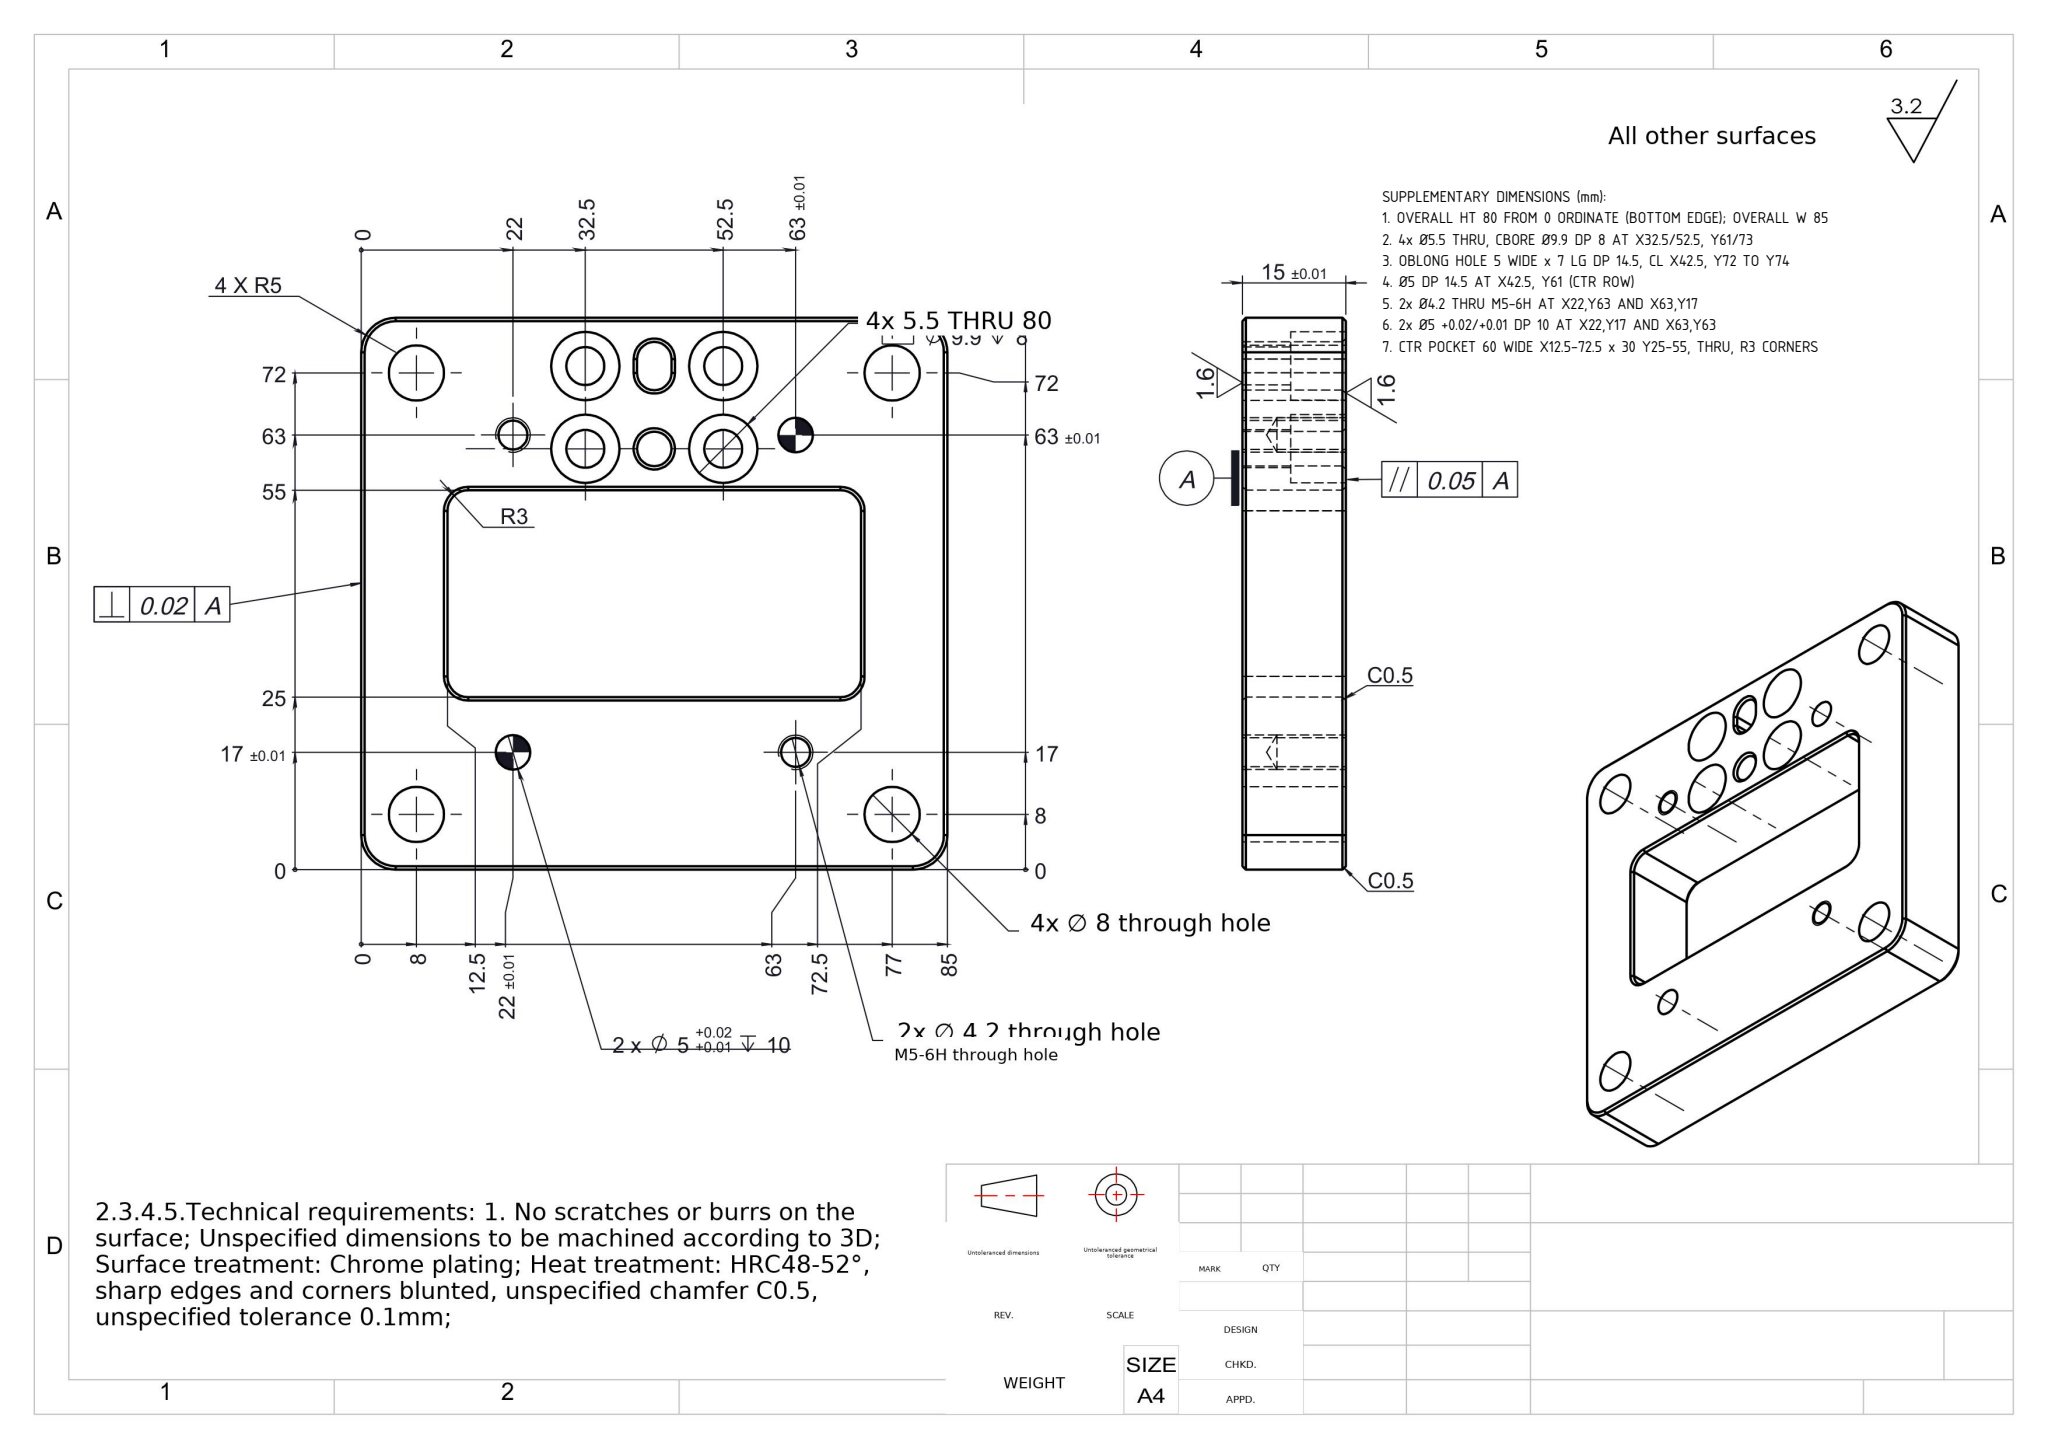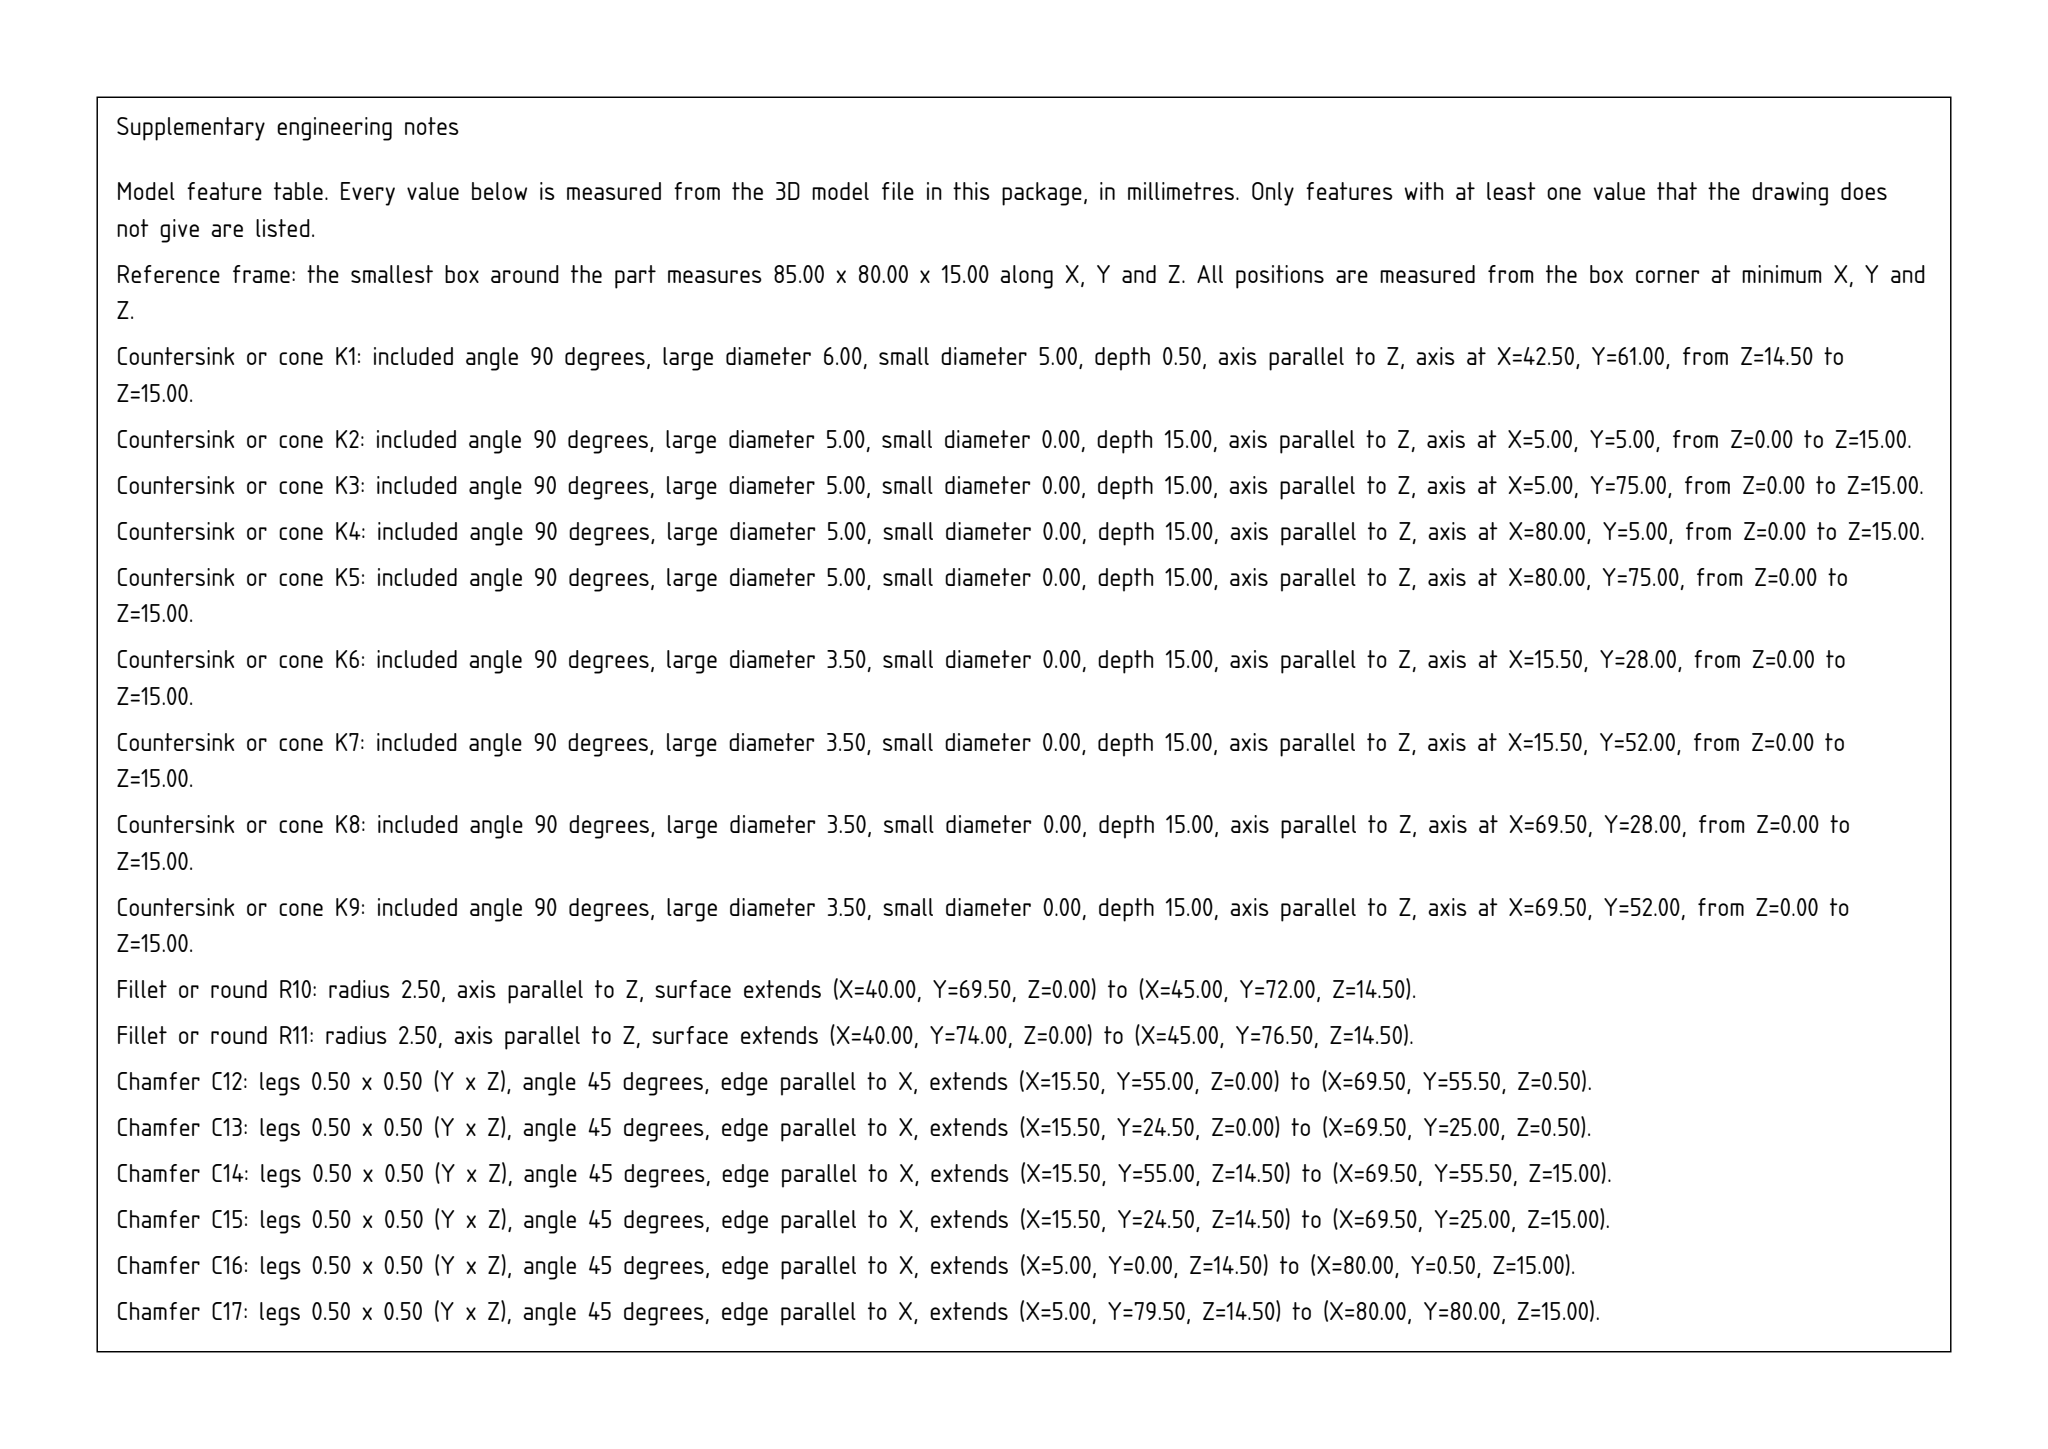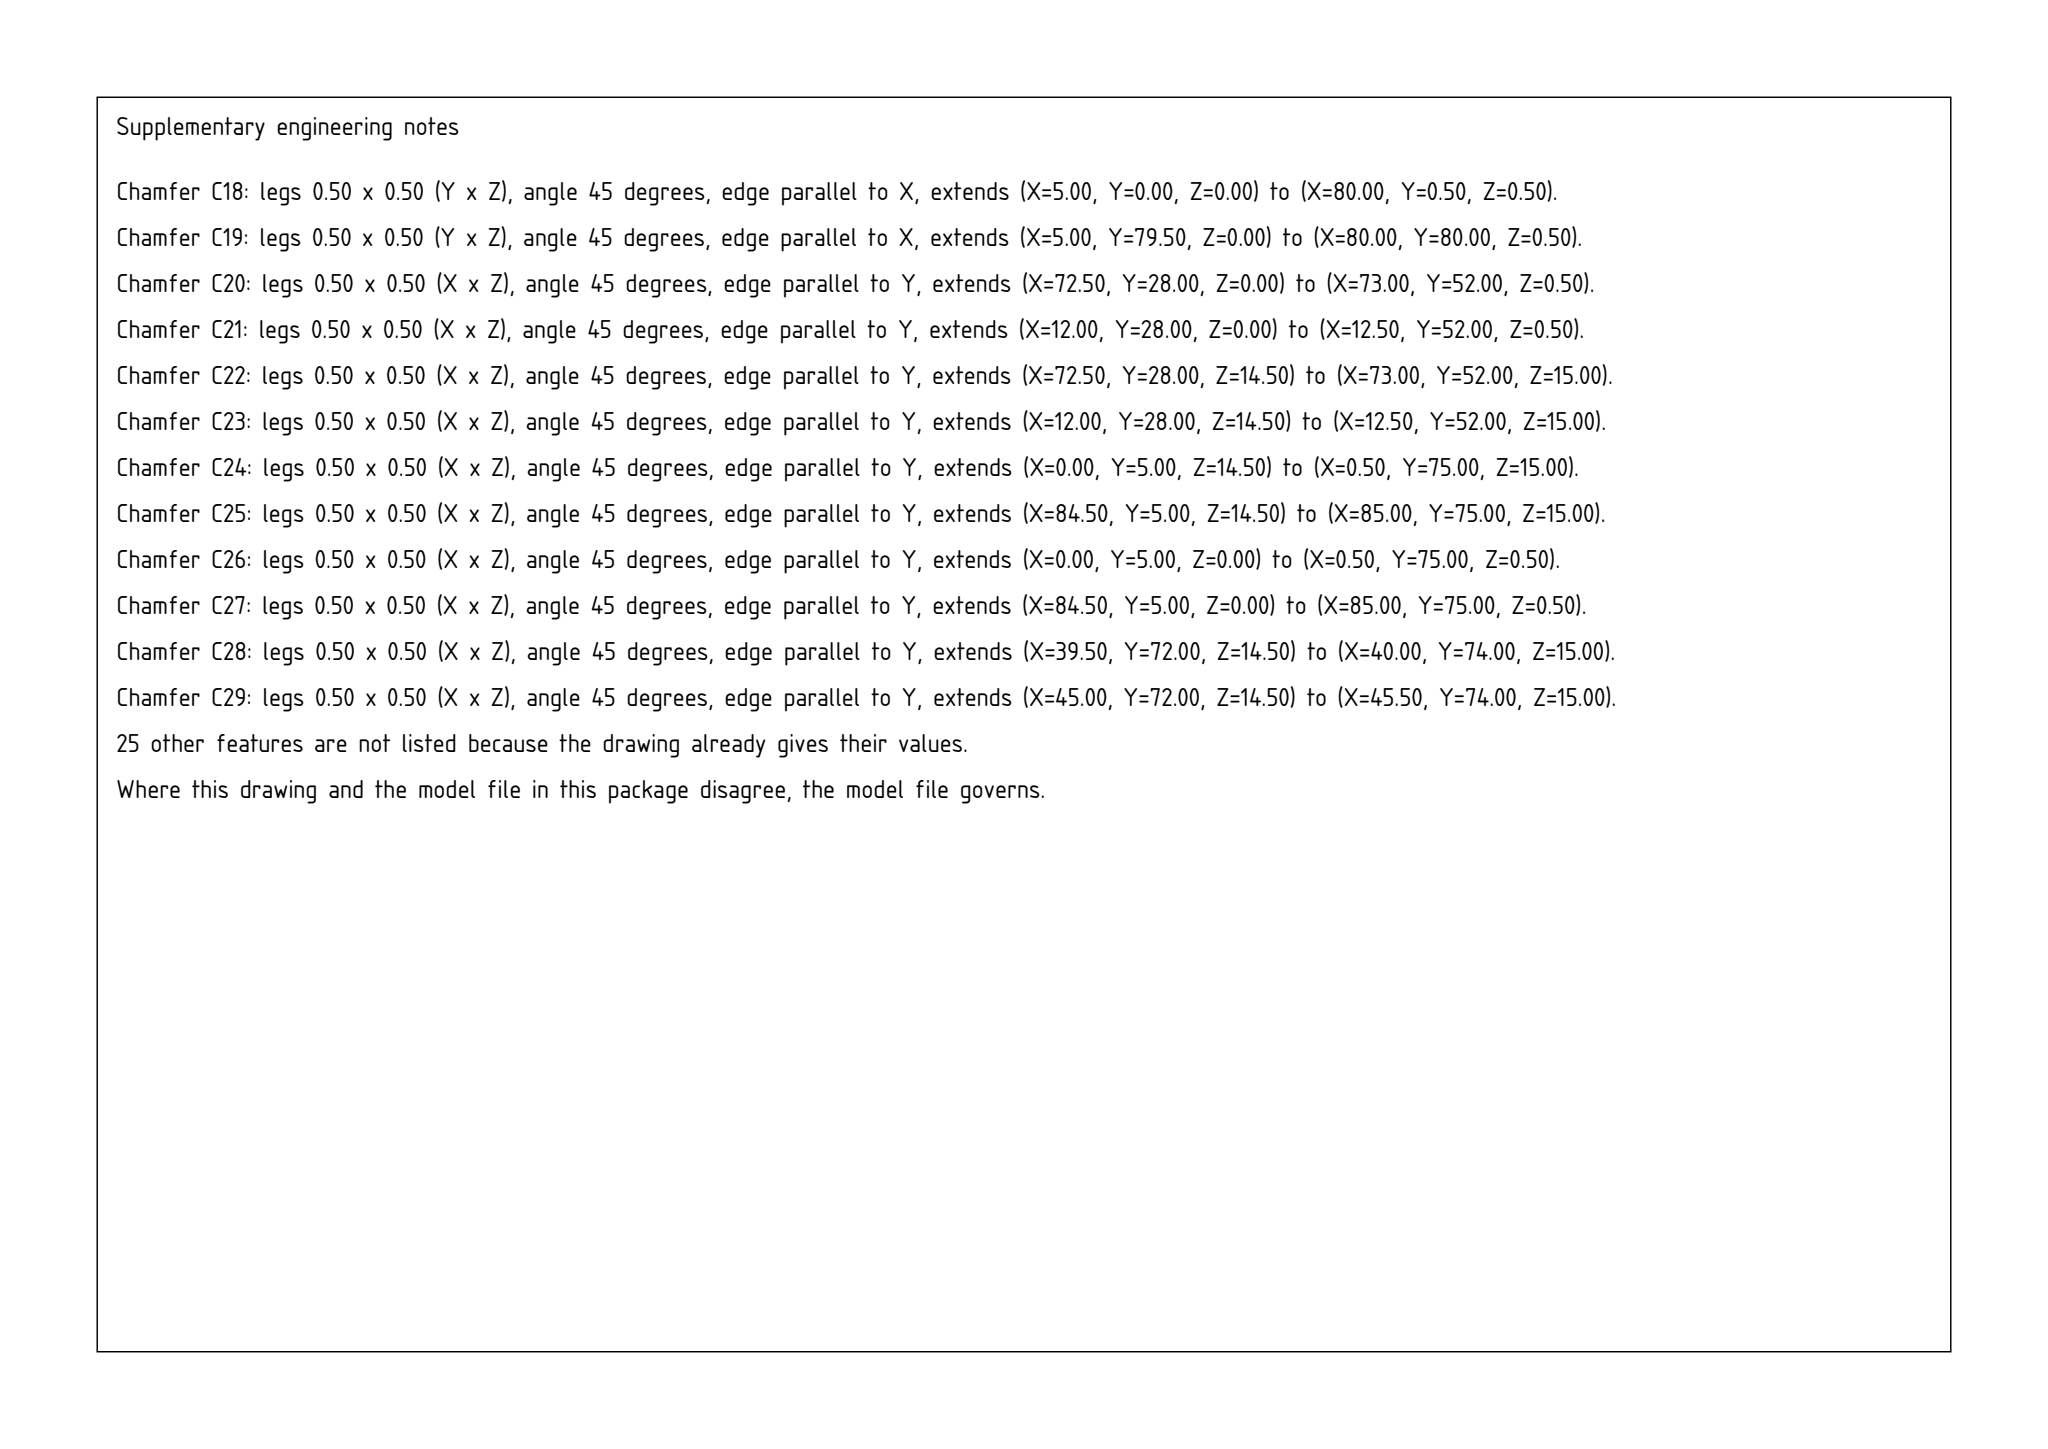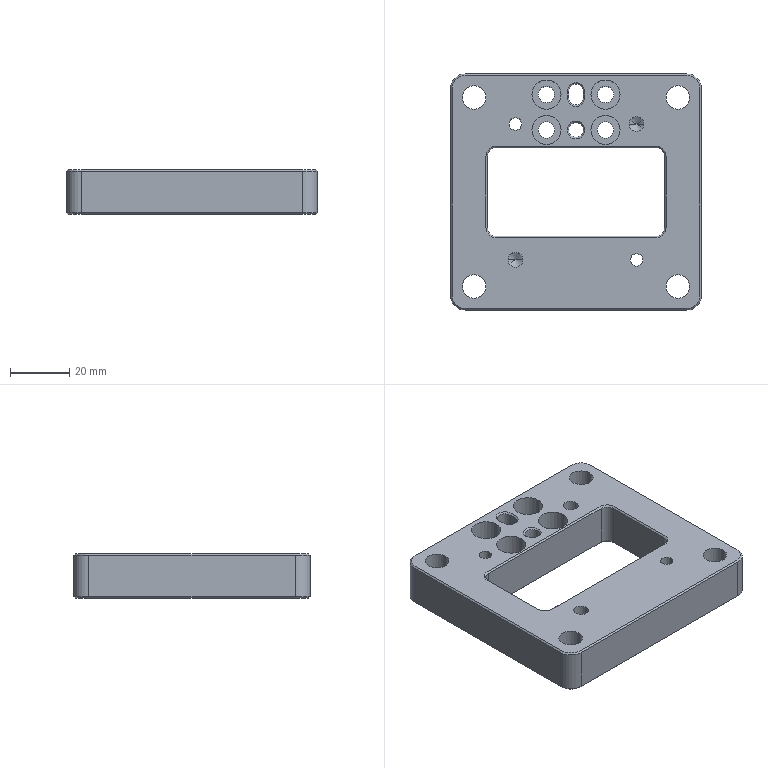Part | SolidWorks | mm | 1 solid | 102 faces | box 85 x 80 x 15 mm | volume 66954 mm3 | cylinder 44 | plane 34 | cone 24 | commonest cylinder face diameters 5 x8 9.9 x8 5.5 x8 8 x8 4.2 x4 10 x4 6 x4